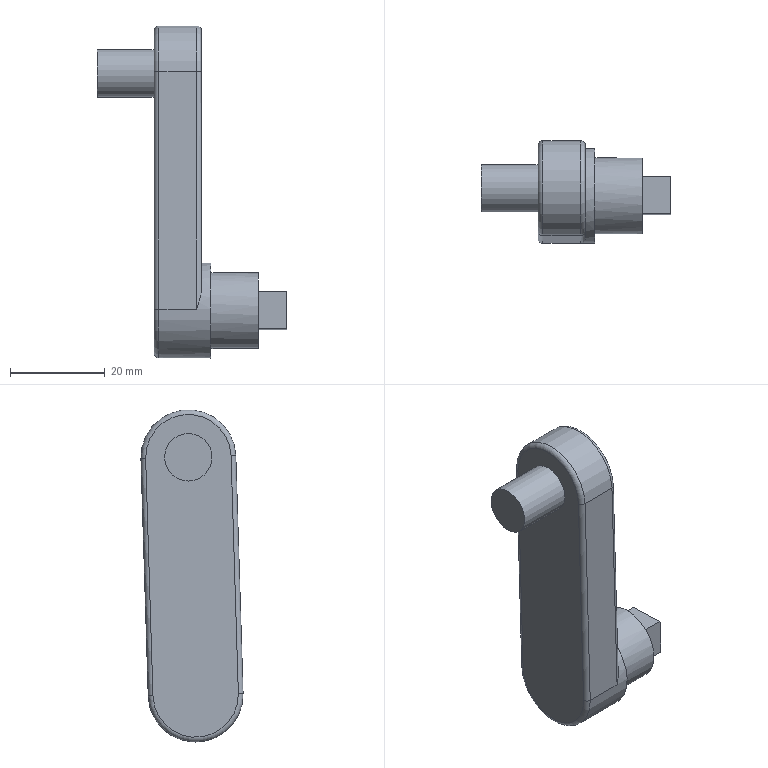Component | NX | ROCKER | 1 solid | 23 faces | volume 17026 mm3 | plane 12 | cylinder 8 | torus 3 | commonest cylinder face diameters 2 x4 20 x2 10 x1 16 x1